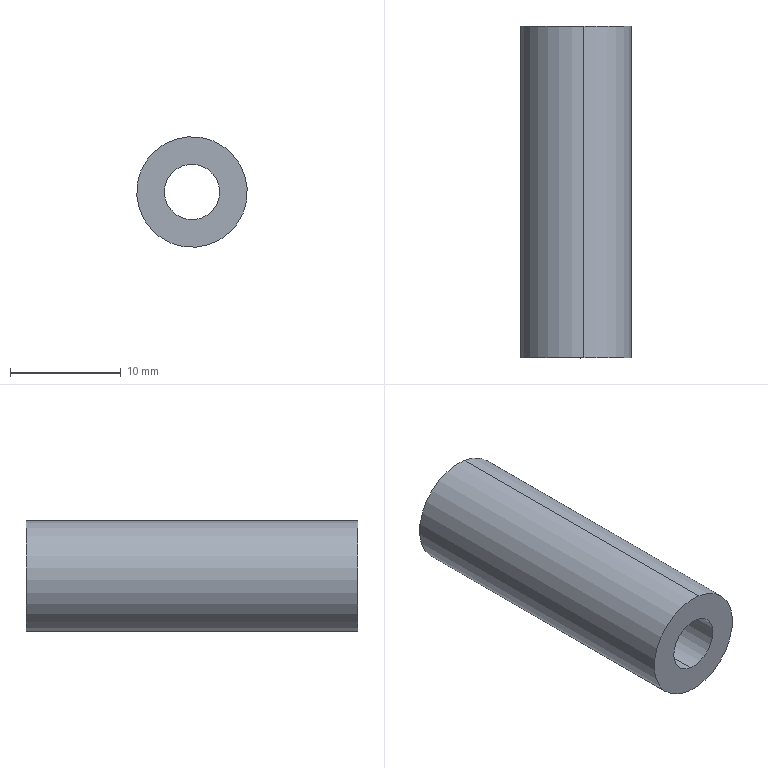Component | SolidWorks | OuterFlipStrip-3 | 1 solid | 6 faces | box 10 x 30 x 10 mm | volume 1767 mm3 | cylinder 4 | plane 2 | commonest cylinder face diameters 5 x2 10 x2
build123d program:
from build123d import *

# Parameters (mm, degrees)
SKETCH1_R           = 5
SKETCH1_R_2         = 2.5
BOSS_EXTRUDE1_DEPTH = 30


with BuildPart() as part:
    # Sketch1 → Boss-Extrude1 (new body)
    with BuildSketch(Plane.XY):
        with Locations((-92, 20)):
            Circle(SKETCH1_R)
        with Locations((-92, 20)):
            Circle(SKETCH1_R_2, mode=Mode.SUBTRACT)
    extrude(amount=BOSS_EXTRUDE1_DEPTH)


solid = part.part

# Placed as in the assembly
solid = solid.moved(Location((-438, 130.5, -20), (90, 0, 0)))
STEP:
#1=COLOUR_RGB('',0.7922,0.8196,0.9333);
#2=FILL_AREA_STYLE_COLOUR('',#1);
#3=FILL_AREA_STYLE('',(#2));
#4=SURFACE_STYLE_FILL_AREA(#3);
#5=SURFACE_SIDE_STYLE('',(#4));
#6=SURFACE_STYLE_USAGE(.BOTH.,#5);
#7=PRESENTATION_STYLE_ASSIGNMENT((#6));
#8=CARTESIAN_POINT('',(-20.88,5.138,-0.0974));
#9=VERTEX_POINT('',#8);
#10=CARTESIAN_POINT('',(-20.852,5.138,0.0974));
#11=VERTEX_POINT('',#10);
#12=CARTESIAN_POINT('',(-20.866,5.138,0.));
#13=DIRECTION('',(0.,1.,0.));
#14=DIRECTION('',(0.1442,0.,0.9896));
#15=AXIS2_PLACEMENT_3D('',#12,#13,#14);
#16=CIRCLE('',#15,0.09843);
#17=EDGE_CURVE('',#9,#11,#16,.T.);
#18=ORIENTED_EDGE('',*,*,#17,.T.);
#19=CARTESIAN_POINT('',(-20.852,3.957,0.0974));
#20=VERTEX_POINT('',#19);
#21=CARTESIAN_POINT('',(-20.852,5.138,0.0974));
#22=DIRECTION('',(-0.,-1.,-0.));
#23=VECTOR('',#22,39.37);
#24=LINE('',#21,#23);
#25=EDGE_CURVE('',#11,#20,#24,.T.);
#26=ORIENTED_EDGE('',*,*,#25,.T.);
#27=CARTESIAN_POINT('',(-20.88,3.957,-0.0974));
#28=VERTEX_POINT('',#27);
#29=CARTESIAN_POINT('',(-20.866,3.957,0.));
#30=DIRECTION('',(0.,1.,0.));
#31=DIRECTION('',(0.1442,-0.,0.9896));
#32=AXIS2_PLACEMENT_3D('',#29,#30,#31);
#33=CIRCLE('',#32,0.09843);
#34=EDGE_CURVE('',#28,#20,#33,.T.);
#35=ORIENTED_EDGE('',*,*,#34,.F.);
#36=CARTESIAN_POINT('',(-20.88,5.138,-0.0974));
#37=DIRECTION('',(-0.,-1.,-0.));
#38=VECTOR('',#37,39.37);
#39=LINE('',#36,#38);
#40=EDGE_CURVE('',#9,#28,#39,.T.);
#41=ORIENTED_EDGE('',*,*,#40,.F.);
#42=EDGE_LOOP('',(#18,#26,#35,#41));
#43=FACE_OUTER_BOUND('',#42,.T.);
#44=CARTESIAN_POINT('',(-20.866,5.138,0.));
#45=DIRECTION('',(-0.,-1.,-0.));
#46=DIRECTION('',(-0.1442,0.,-0.9896));
#47=AXIS2_PLACEMENT_3D('',#44,#45,#46);
#48=CYLINDRICAL_SURFACE('',#47,0.09843);
#49=ADVANCED_FACE('',(#43),#48,.F.);
#50=CARTESIAN_POINT('',(-20.838,5.138,0.1948));
#51=VERTEX_POINT('',#50);
#52=CARTESIAN_POINT('',(-20.895,5.138,-0.1948));
#53=VERTEX_POINT('',#52);
#54=CARTESIAN_POINT('',(-20.866,5.138,0.));
#55=DIRECTION('',(0.,1.,0.));
#56=DIRECTION('',(0.1442,-0.,0.9896));
#57=AXIS2_PLACEMENT_3D('',#54,#55,#56);
#58=CIRCLE('',#57,0.1969);
#59=EDGE_CURVE('',#51,#53,#58,.T.);
#60=ORIENTED_EDGE('',*,*,#59,.F.);
#61=CARTESIAN_POINT('',(-20.838,3.957,0.1948));
#62=VERTEX_POINT('',#61);
#63=CARTESIAN_POINT('',(-20.838,5.138,0.1948));
#64=DIRECTION('',(-0.,-1.,-0.));
#65=VECTOR('',#64,39.37);
#66=LINE('',#63,#65);
#67=EDGE_CURVE('',#51,#62,#66,.T.);
#68=ORIENTED_EDGE('',*,*,#67,.T.);
#69=CARTESIAN_POINT('',(-20.895,3.957,-0.1948));
#70=VERTEX_POINT('',#69);
#71=CARTESIAN_POINT('',(-20.866,3.957,0.));
#72=DIRECTION('',(0.,1.,0.));
#73=DIRECTION('',(0.1442,-0.,0.9896));
#74=AXIS2_PLACEMENT_3D('',#71,#72,#73);
#75=CIRCLE('',#74,0.1969);
#76=EDGE_CURVE('',#62,#70,#75,.T.);
#77=ORIENTED_EDGE('',*,*,#76,.T.);
#78=CARTESIAN_POINT('',(-20.895,5.138,-0.1948));
#79=DIRECTION('',(-0.,-1.,-0.));
#80=VECTOR('',#79,39.37);
#81=LINE('',#78,#80);
#82=EDGE_CURVE('',#53,#70,#81,.T.);
#83=ORIENTED_EDGE('',*,*,#82,.F.);
#84=EDGE_LOOP('',(#60,#68,#77,#83));
#85=FACE_OUTER_BOUND('',#84,.T.);
#86=CARTESIAN_POINT('',(-20.866,5.138,0.));
#87=DIRECTION('',(-0.,-1.,-0.));
#88=DIRECTION('',(-0.1442,0.,-0.9896));
#89=AXIS2_PLACEMENT_3D('',#86,#87,#88);
#90=CYLINDRICAL_SURFACE('',#89,0.1969);
#91=ADVANCED_FACE('',(#85),#90,.T.);
#92=CARTESIAN_POINT('',(-20.866,5.138,0.));
#93=DIRECTION('',(0.,1.,0.));
#94=DIRECTION('',(0.1442,-0.,0.9896));
#95=AXIS2_PLACEMENT_3D('',#92,#93,#94);
#96=CIRCLE('',#95,0.1969);
#97=EDGE_CURVE('',#53,#51,#96,.T.);
#98=ORIENTED_EDGE('',*,*,#97,.T.);
#99=ORIENTED_EDGE('',*,*,#59,.T.);
#100=EDGE_LOOP('',(#98,#99));
#101=FACE_OUTER_BOUND('',#100,.T.);
#102=ORIENTED_EDGE('',*,*,#17,.F.);
#103=CARTESIAN_POINT('',(-20.866,5.138,0.));
#104=DIRECTION('',(0.,1.,0.));
#105=DIRECTION('',(0.1442,0.,0.9896));
#106=AXIS2_PLACEMENT_3D('',#103,#104,#105);
#107=CIRCLE('',#106,0.09843);
#108=EDGE_CURVE('',#11,#9,#107,.T.);
#109=ORIENTED_EDGE('',*,*,#108,.F.);
#110=EDGE_LOOP('',(#102,#109));
#111=FACE_BOUND('',#110,.T.);
#112=CARTESIAN_POINT('',(-20.866,5.138,0.));
#113=DIRECTION('',(0.,1.,0.));
#114=DIRECTION('',(0.1442,-0.,0.9896));
#115=AXIS2_PLACEMENT_3D('',#112,#113,#114);
#116=PLANE('',#115);
#117=ADVANCED_FACE('',(#101,#111),#116,.T.);
#118=CARTESIAN_POINT('',(-20.866,3.957,0.));
#119=DIRECTION('',(0.,1.,0.));
#120=DIRECTION('',(0.1442,-0.,0.9896));
#121=AXIS2_PLACEMENT_3D('',#118,#119,#120);
#122=CIRCLE('',#121,0.1969);
#123=EDGE_CURVE('',#70,#62,#122,.T.);
#124=ORIENTED_EDGE('',*,*,#123,.F.);
#125=ORIENTED_EDGE('',*,*,#76,.F.);
#126=EDGE_LOOP('',(#124,#125));
#127=FACE_OUTER_BOUND('',#126,.T.);
#128=ORIENTED_EDGE('',*,*,#34,.T.);
#129=CARTESIAN_POINT('',(-20.866,3.957,0.));
#130=DIRECTION('',(0.,1.,0.));
#131=DIRECTION('',(0.1442,-0.,0.9896));
#132=AXIS2_PLACEMENT_3D('',#129,#130,#131);
#133=CIRCLE('',#132,0.09843);
#134=EDGE_CURVE('',#20,#28,#133,.T.);
#135=ORIENTED_EDGE('',*,*,#134,.T.);
#136=EDGE_LOOP('',(#128,#135));
#137=FACE_BOUND('',#136,.T.);
#138=CARTESIAN_POINT('',(-20.866,3.957,0.));
#139=DIRECTION('',(0.,1.,0.));
#140=DIRECTION('',(0.1442,-0.,0.9896));
#141=AXIS2_PLACEMENT_3D('',#138,#139,#140);
#142=PLANE('',#141);
#143=ADVANCED_FACE('',(#127,#137),#142,.F.);
#144=ORIENTED_EDGE('',*,*,#67,.F.);
#145=ORIENTED_EDGE('',*,*,#97,.F.);
#146=ORIENTED_EDGE('',*,*,#82,.T.);
#147=ORIENTED_EDGE('',*,*,#123,.T.);
#148=EDGE_LOOP('',(#144,#145,#146,#147));
#149=FACE_OUTER_BOUND('',#148,.T.);
#150=CARTESIAN_POINT('',(-20.866,5.138,0.));
#151=DIRECTION('',(-0.,-1.,-0.));
#152=DIRECTION('',(-0.1442,0.,-0.9896));
#153=AXIS2_PLACEMENT_3D('',#150,#151,#152);
#154=CYLINDRICAL_SURFACE('',#153,0.1969);
#155=ADVANCED_FACE('',(#149),#154,.T.);
#156=ORIENTED_EDGE('',*,*,#25,.F.);
#157=ORIENTED_EDGE('',*,*,#108,.T.);
#158=ORIENTED_EDGE('',*,*,#40,.T.);
#159=ORIENTED_EDGE('',*,*,#134,.F.);
#160=EDGE_LOOP('',(#156,#157,#158,#159));
#161=FACE_OUTER_BOUND('',#160,.T.);
#162=CARTESIAN_POINT('',(-20.866,5.138,0.));
#163=DIRECTION('',(-0.,-1.,-0.));
#164=DIRECTION('',(-0.1442,0.,-0.9896));
#165=AXIS2_PLACEMENT_3D('',#162,#163,#164);
#166=CYLINDRICAL_SURFACE('',#165,0.09843);
#167=ADVANCED_FACE('',(#161),#166,.F.);
#168=CLOSED_SHELL('',(#49,#91,#117,#143,#155,#167));
#169=MANIFOLD_SOLID_BREP('',#168);
#170=STYLED_ITEM('',(#7),#169);
#171=PRESENTATION_LAYER_ASSIGNMENT('','',(#170));
#172=(LENGTH_UNIT()NAMED_UNIT(*)SI_UNIT($,.METRE.));
#173=LENGTH_MEASURE_WITH_UNIT(LENGTH_MEASURE(0.0254),#172);
#174=DIMENSIONAL_EXPONENTS(1.,0.,0.,0.,0.,0.,0.);
#175=(CONVERSION_BASED_UNIT('',#173)LENGTH_UNIT()NAMED_UNIT(#174));
#176=UNCERTAINTY_MEASURE_WITH_UNIT(LENGTH_MEASURE(0.00001),#175,'','');
#177=(NAMED_UNIT(*)PLANE_ANGLE_UNIT()SI_UNIT($,.RADIAN.));
#178=(NAMED_UNIT(*)SI_UNIT($,.STERADIAN.)SOLID_ANGLE_UNIT());
#179=(GEOMETRIC_REPRESENTATION_CONTEXT(3)GLOBAL_UNCERTAINTY_ASSIGNED_CONTEXT((#176))GLOBAL_UNIT_ASSIGNED_CONTEXT((#175,#177,#178))REPRESENTATION_CONTEXT('',''));
#180=MECHANICAL_DESIGN_GEOMETRIC_PRESENTATION_REPRESENTATION('',(#170),#179);
#181=CARTESIAN_POINT('',(0.,0.,0.));
#182=DIRECTION('',(0.,0.,1.));
#183=DIRECTION('',(1.,0.,0.));
#184=AXIS2_PLACEMENT_3D('',#181,#182,#183);
#185=(LENGTH_UNIT()NAMED_UNIT(*)SI_UNIT($,.METRE.));
#186=LENGTH_MEASURE_WITH_UNIT(LENGTH_MEASURE(0.0254),#185);
#187=DIMENSIONAL_EXPONENTS(1.,0.,0.,0.,0.,0.,0.);
#188=(CONVERSION_BASED_UNIT('',#186)LENGTH_UNIT()NAMED_UNIT(#187));
#189=UNCERTAINTY_MEASURE_WITH_UNIT(LENGTH_MEASURE(0.00001),#188,'','');
#190=(NAMED_UNIT(*)PLANE_ANGLE_UNIT()SI_UNIT($,.RADIAN.));
#191=(NAMED_UNIT(*)SI_UNIT($,.STERADIAN.)SOLID_ANGLE_UNIT());
#192=(GEOMETRIC_REPRESENTATION_CONTEXT(3)GLOBAL_UNCERTAINTY_ASSIGNED_CONTEXT((#189))GLOBAL_UNIT_ASSIGNED_CONTEXT((#188,#190,#191))REPRESENTATION_CONTEXT('',''));
#193=ADVANCED_BREP_SHAPE_REPRESENTATION('',(#169,#184),#192);